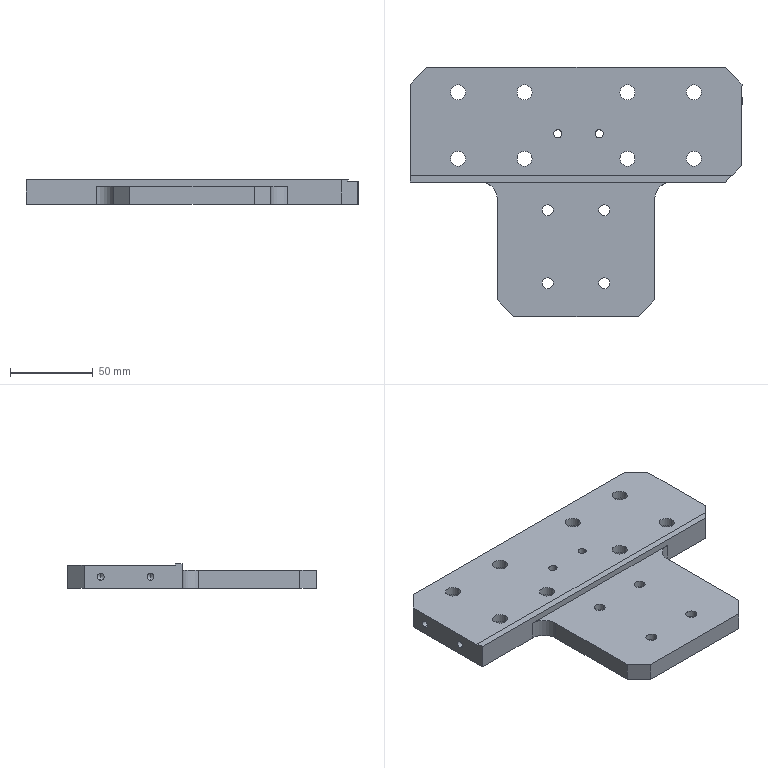Component | SolidWorks | LongSideClampingAssemblyBGeneralAssembly-1_ClampingMountingPlateB-0510-1 | 1 solid | 99 faces | box 200 x 150 x 15 mm | volume 255920 mm3 | cylinder 62 | plane 29 | cone 8 | commonest cylinder face diameters 15 x16 9 x16 4.2 x8 11 x8 6.6 x8 5 x4 20 x2 | material Q235-A
build123d program:
from build123d import *

# Parameters (mm, degrees)
SKETCH1_W                                          = 200
SKETCH1_H                                          = 150
BOSS_EXTRUDE1_DEPTH                                = 15
HOLE_SIZE_ACCORDING_TO_TYPE_OF_HEX_SOC_D           = 9
HOLE_SIZE_ACCORDING_TO_TYPE_OF_HEX_SOC_CBORE_D     = 15
HOLE_SIZE_ACCORDING_TO_TYPE_OF_HEX_SOC_CBORE_DEPTH = 9
SKETCH10_W                                         = 200
SKETCH10_H                                         = 81
CUT_EXTRUDE2_DEPTH                                 = 4
HOLE_SIZE_ACCORDING_TO_TYPE_OF_HEX_2_D             = 6.6
HOLE_SIZE_ACCORDING_TO_TYPE_OF_HEX_2_CBORE_D       = 11
HOLE_SIZE_ACCORDING_TO_TYPE_OF_HEX_2_CBORE_DEPTH   = 6.8
SKETCH13_W                                         = 200
SKETCH13_H                                         = 65
CUT_EXTRUDE3_DEPTH                                 = 1
SKETCH14_W                                         = 52.5
SKETCH14_H                                         = 81
CUT_EXTRUDE4_DEPTH                                 = 251.45
FILLET1_R                                          = 10
CHAMFER1_SIZE                                      = 10
M6_TAPPED_HOLE1_D                                  = 5
M5_TAPPED_HOLE1_AT_2_COUNT                         = 2
M5_TAPPED_HOLE1_AT_2_PITCH                         = 30


with BuildPart() as part:
    # Sketch1 → Boss-Extrude1 (new body)
    with BuildSketch(Plane(origin=(0, 0, 0), x_dir=(0, 0, -1), z_dir=(1, 0, 0))):
        with Locations((100, -75)):
            Rectangle(SKETCH1_W, SKETCH1_H)
    extrude(amount=BOSS_EXTRUDE1_DEPTH)

    # Hole Size _According to_ Type of Hex Soc (through all)
    with Locations(Plane(origin=(15, 0, 0), x_dir=(0, 0, -1), z_dir=(1, 0, 0))):
        with Locations((29, -15), (29, -55), (69, -55), (69, -15), (131, -55), (131, -15), (171, -15), (171, -55)):
            CounterBoreHole(HOLE_SIZE_ACCORDING_TO_TYPE_OF_HEX_SOC_D / 2, HOLE_SIZE_ACCORDING_TO_TYPE_OF_HEX_SOC_CBORE_D / 2, HOLE_SIZE_ACCORDING_TO_TYPE_OF_HEX_SOC_CBORE_DEPTH)

    # Sketch10 → Cut-Extrude2 (cut)
    with BuildSketch(Plane.ZY):
        with Locations((-100, -109.5)):
            Rectangle(SKETCH10_W, SKETCH10_H)
    extrude(amount=-CUT_EXTRUDE2_DEPTH, mode=Mode.SUBTRACT)

    # Hole Size _According to_ Type of Hex 2 (through all)
    with Locations(Plane(origin=(15, 0, 0), x_dir=(0, 0, -1), z_dir=(1, 0, 0))):
        with Locations((117, -130), (83, -130), (117, -86), (83, -86)):
            CounterBoreHole(HOLE_SIZE_ACCORDING_TO_TYPE_OF_HEX_2_D / 2, HOLE_SIZE_ACCORDING_TO_TYPE_OF_HEX_2_CBORE_D / 2, HOLE_SIZE_ACCORDING_TO_TYPE_OF_HEX_2_CBORE_DEPTH)

    # Sketch13 → Cut-Extrude3 (cut)
    with BuildSketch(Plane.ZY):
        with Locations((-100, -32.5)):
            Rectangle(SKETCH13_W, SKETCH13_H)
    extrude(amount=-CUT_EXTRUDE3_DEPTH, mode=Mode.SUBTRACT)

    # Sketch14 → Cut-Extrude4 (cut, through all)
    with BuildSketch(Plane(origin=(15, 0, 0), x_dir=(0, 0, -1), z_dir=(1, 0, 0))):
        with Locations((26.25, -109.5)):
            Rectangle(SKETCH14_W, SKETCH14_H)
        with Locations((173.75, -109.5)):
            Rectangle(SKETCH14_W, SKETCH14_H)
    extrude(amount=-CUT_EXTRUDE4_DEPTH, mode=Mode.SUBTRACT)

    # Fillet1
    fillet1_edges = [part.edges().sort_by_distance(p)[0] for p in [
        (9.5, -69, -52.5),
        (9.5, -69, -147.5),
    ]]
    fillet(fillet1_edges, radius=FILLET1_R)

    # Chamfer1
    chamfer1_edges = [part.edges().sort_by_distance(p)[0] for p in [
        (8, 0, -200),
        (8, 0, 0),
        (7.5, -69, 0),
        (9.5, -150, -52.5),
        (9.5, -150, -147.5),
    ]]
    chamfer(chamfer1_edges, length=CHAMFER1_SIZE)

    # M6 Tapped Hole1 (through all)
    with Locations(Plane(origin=(15, 0, 0), x_dir=(0, 0, -1), z_dir=(1, 0, 0))):
        with Locations((85.958, -40), (110.958, -40)):
            Hole(M6_TAPPED_HOLE1_D / 2)

    # Sketch19 → M5 Tapped Hole1 (revolve, cut)
    with BuildSketch(Plane(origin=(8, -20, 0), x_dir=(0, -1, 0), z_dir=(1, 0, 0))):
        Polygon((0, 0), (0, 18.662), (2.1, 17.4), (2.1, 0), align=None)
    m5_tapped_hole1 = revolve(axis=Axis((8, -20, 6.35), (0, 0, -1)), mode=Mode.SUBTRACT)

    # M5 Tapped Hole1 at 2: M5 Tapped Hole1 ×2
    with Locations(*[(0, -i * M5_TAPPED_HOLE1_AT_2_PITCH, 0) for i in range(1, M5_TAPPED_HOLE1_AT_2_COUNT)]):
        add(m5_tapped_hole1, mode=Mode.SUBTRACT)

    # Mirror1: M5 Tapped Hole1 across plane
    add(m5_tapped_hole1.mirror(Plane.XY.offset(-100)), mode=Mode.SUBTRACT)

    # Mirror1 copy 1 sketch → Mirror1 copy 1 (revolve, cut)
    with BuildSketch(Plane(origin=(8, -50, -200), x_dir=(0, -1, 0), z_dir=(1, 0, 0))):
        Polygon((0, 0), (0, -18.662), (2.1, -17.4), (2.1, 0), align=None)
    revolve(axis=Axis((8, -50, -206.35), (0, 0, -1)), mode=Mode.SUBTRACT)


solid = part.part

# Placed as in the assembly
solid = solid.moved(Location((-3020.658, 35.391, 3501.5), (0, 90, 0)))